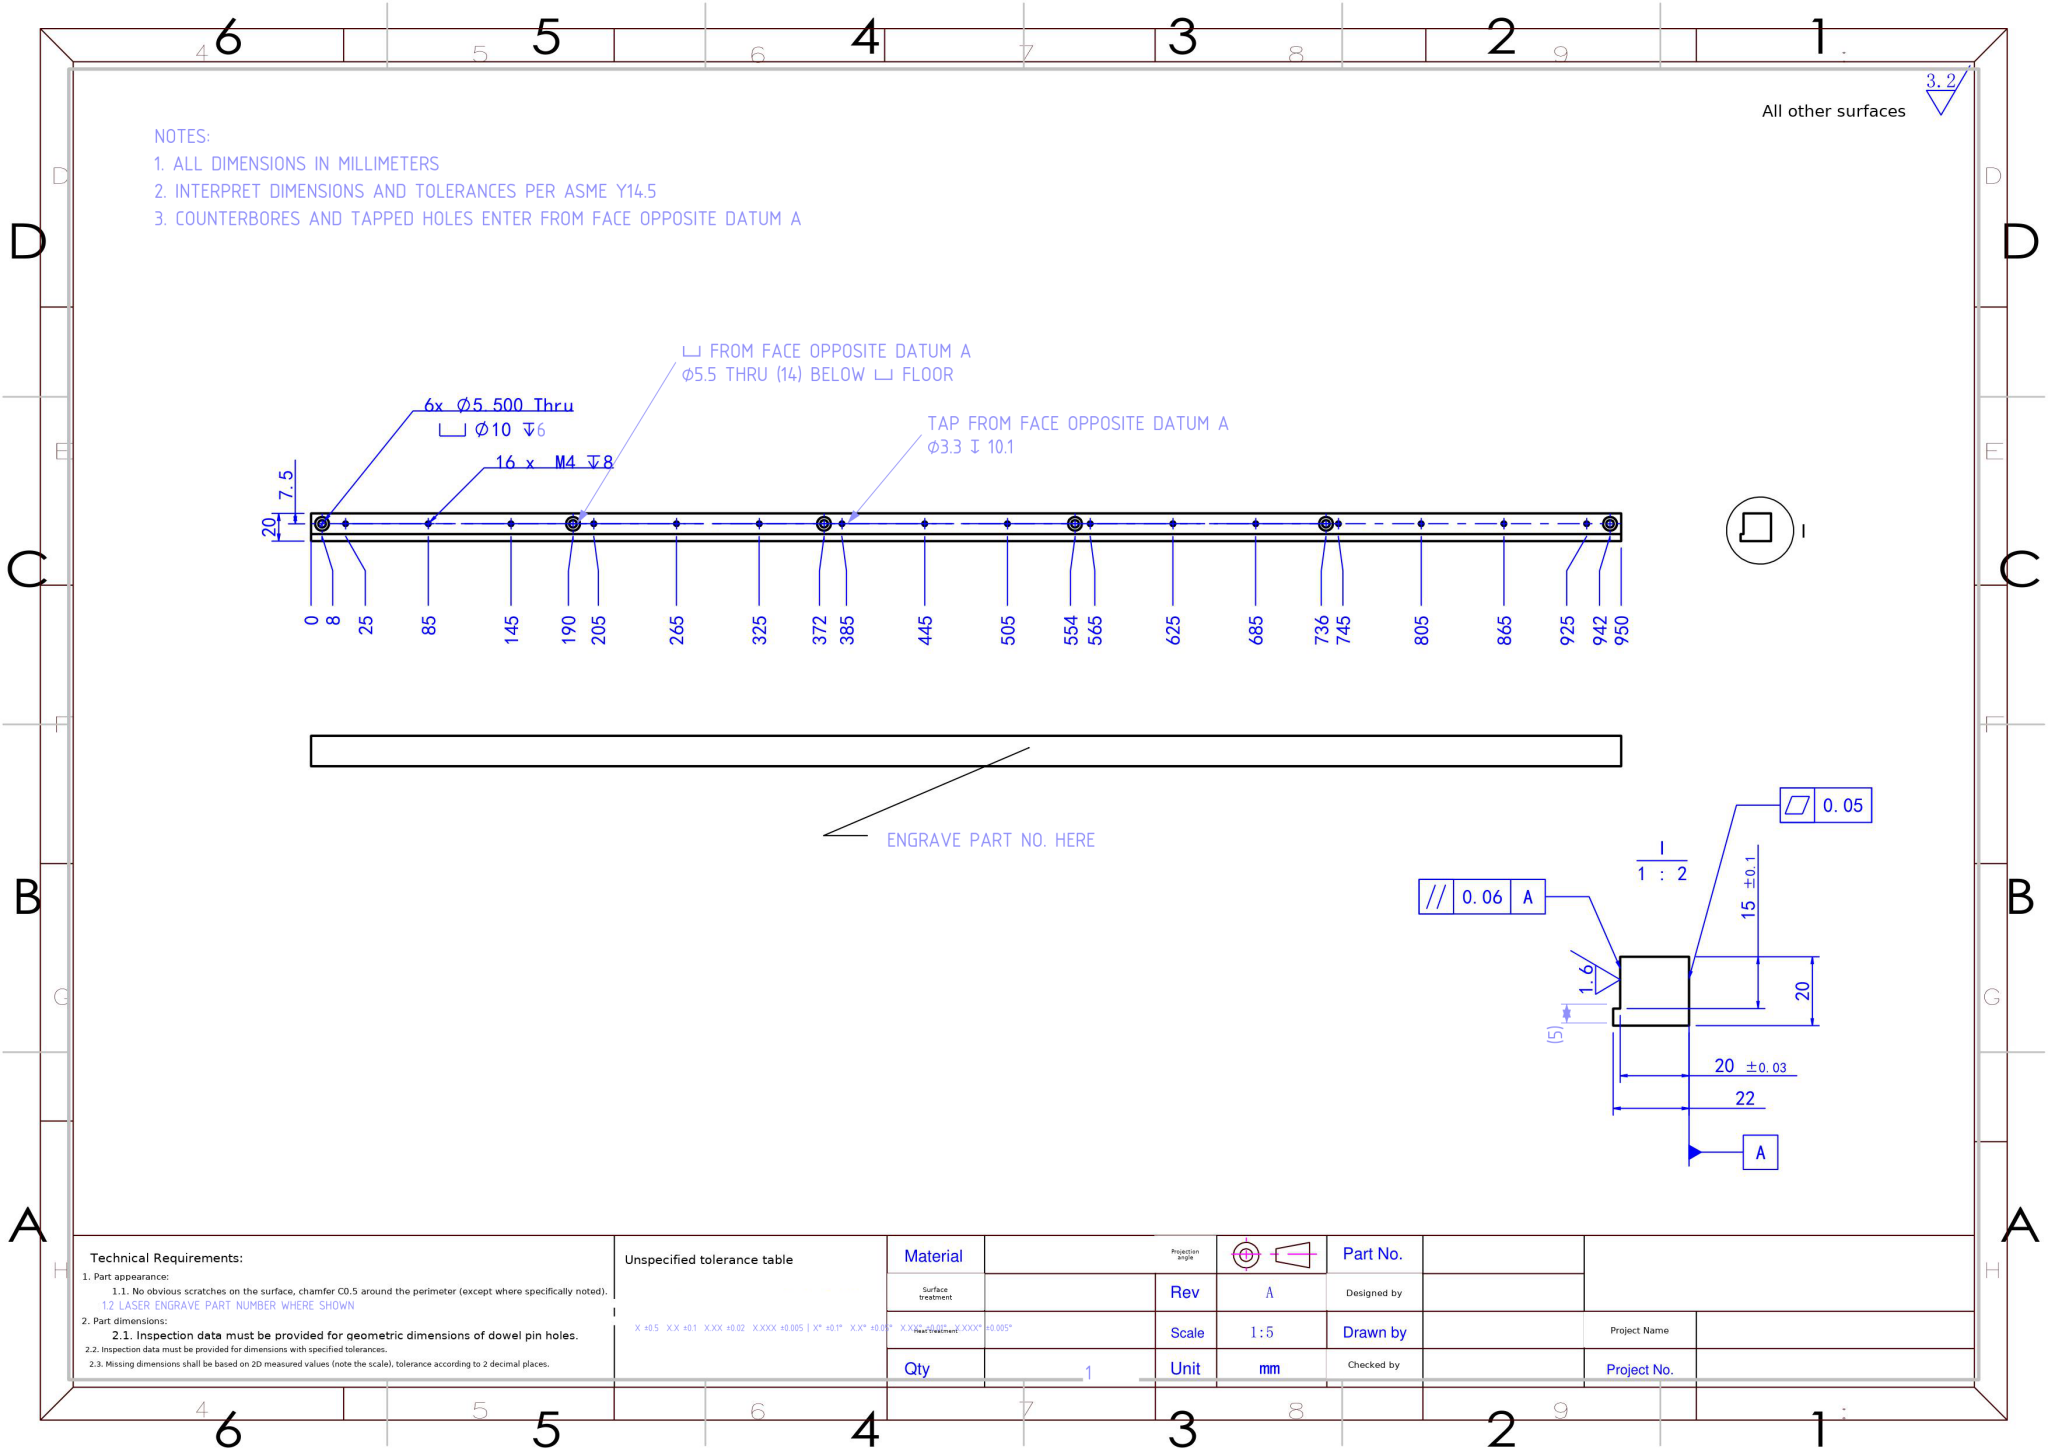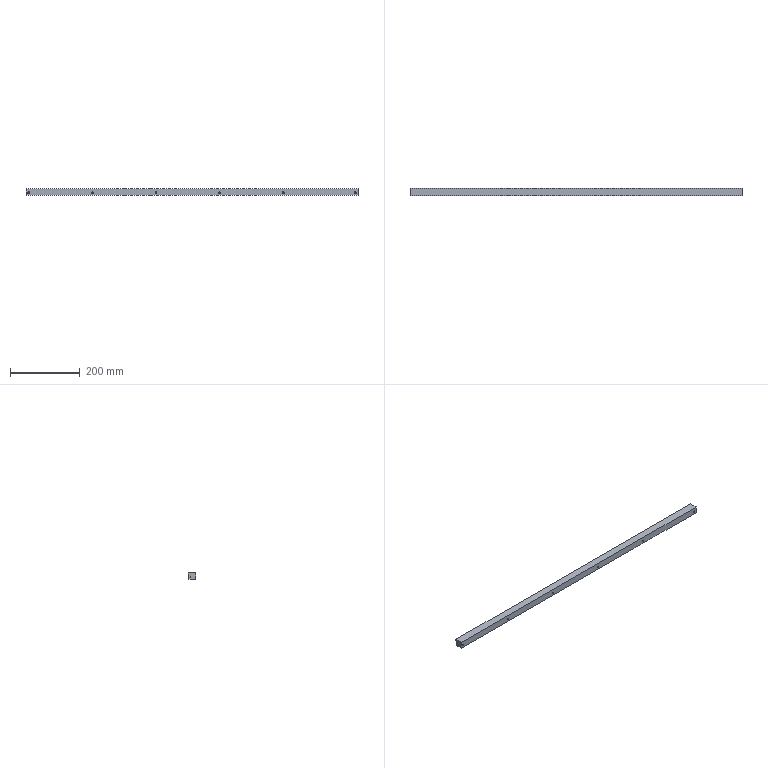Part | NX | mm | 1 solid | 102 faces | box 950 x 22 x 20 mm | volume 383249 mm3 | cylinder 56 | cone 32 | plane 14 | commonest cylinder face diameters 3.3 x32 10 x12 5.5 x12